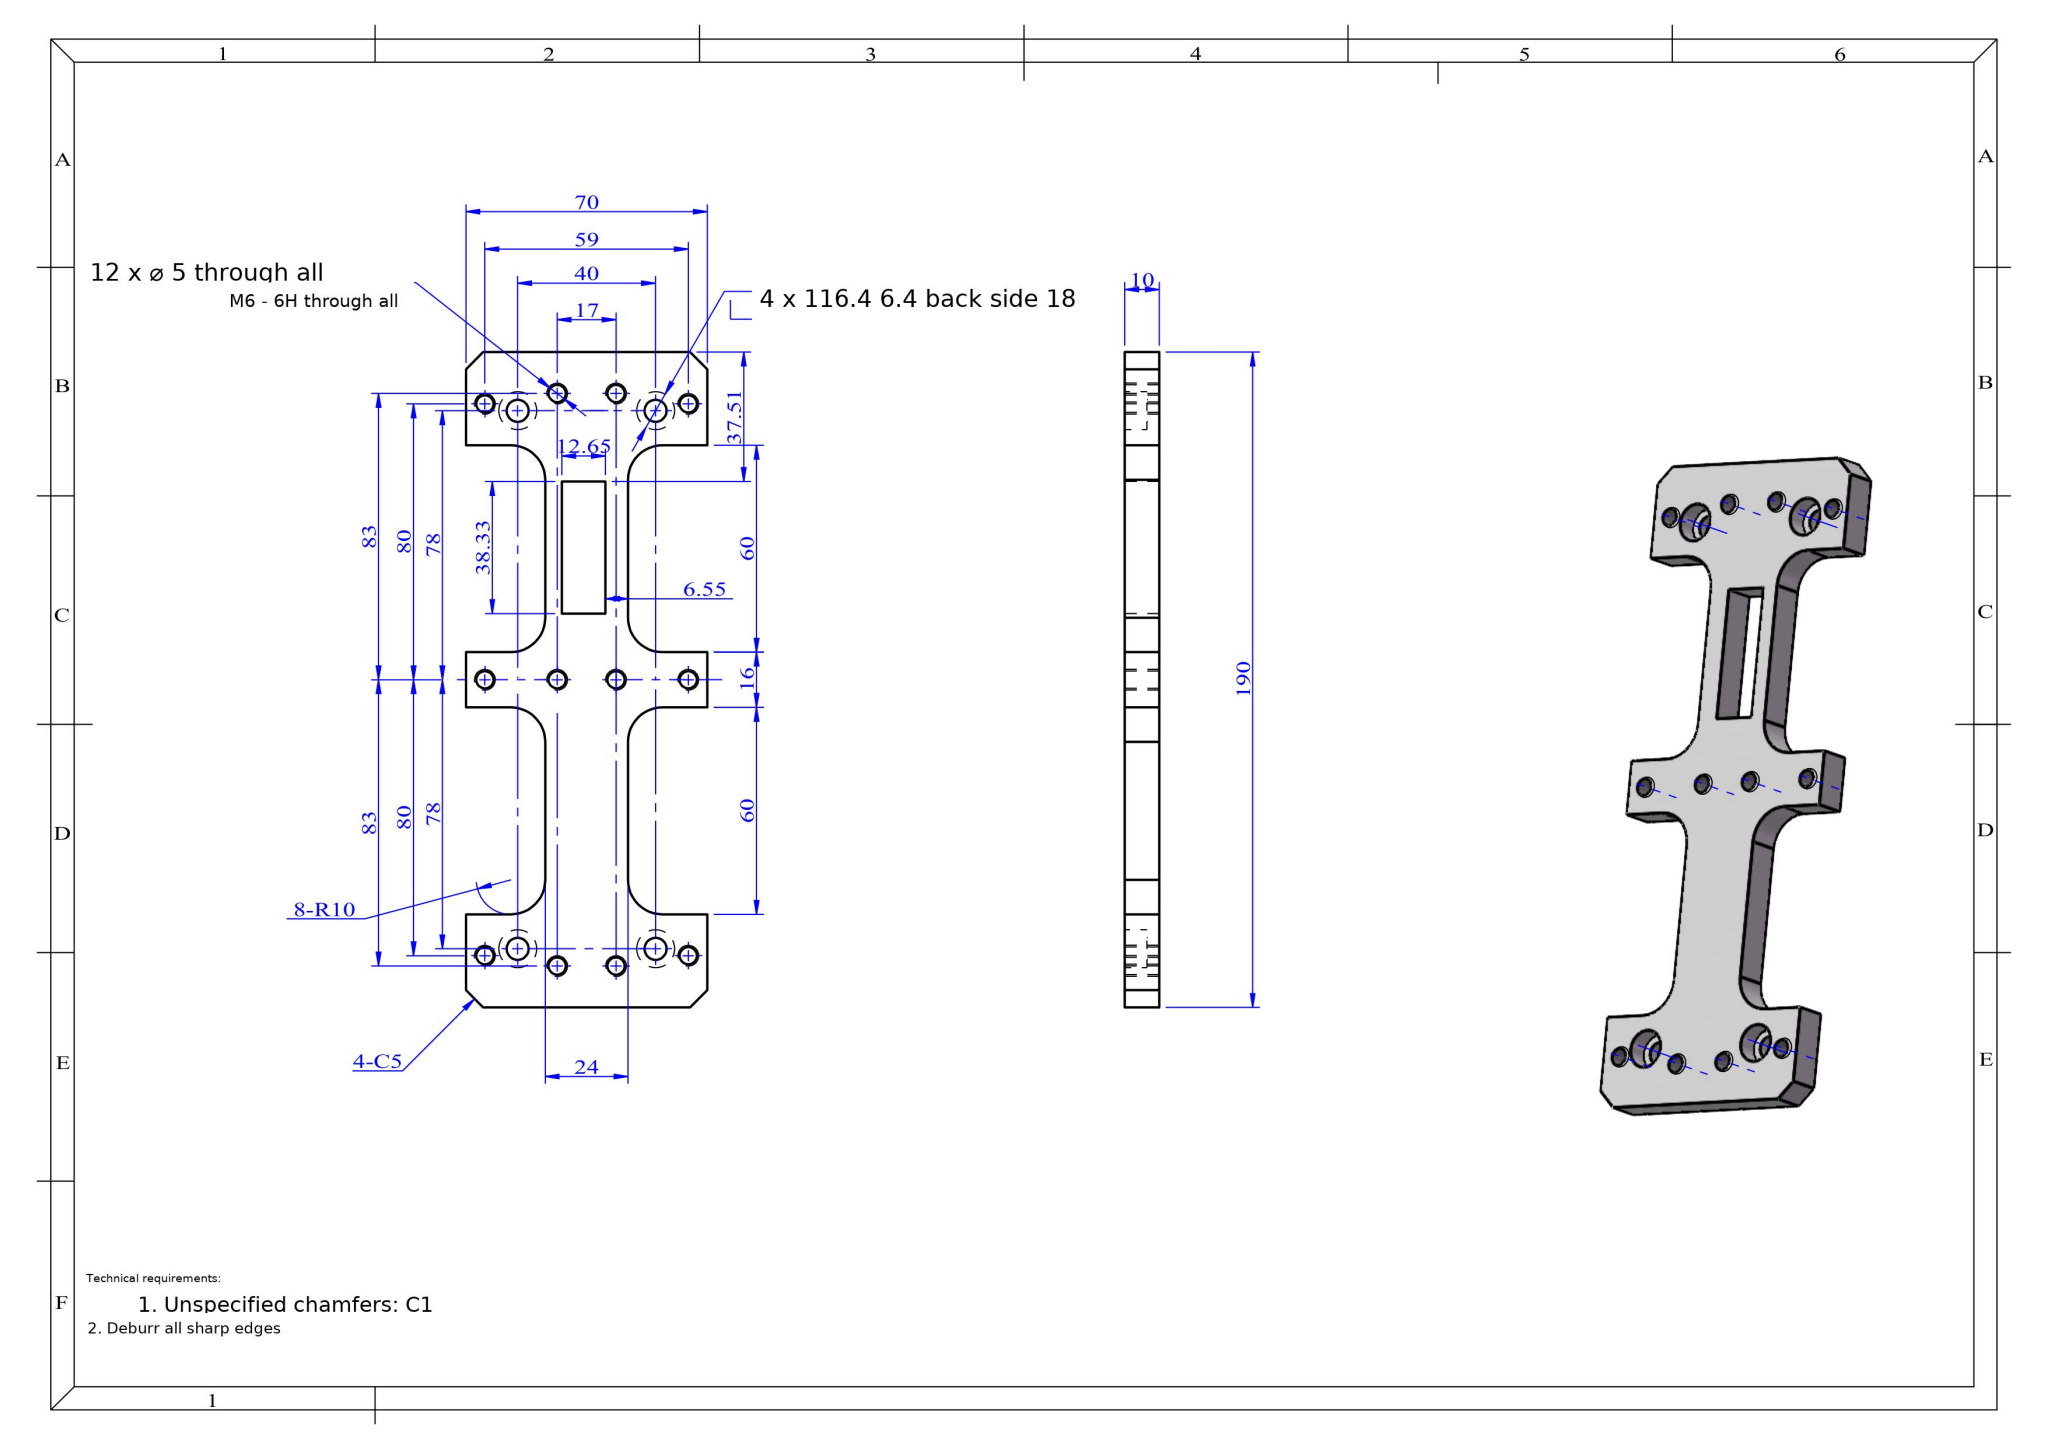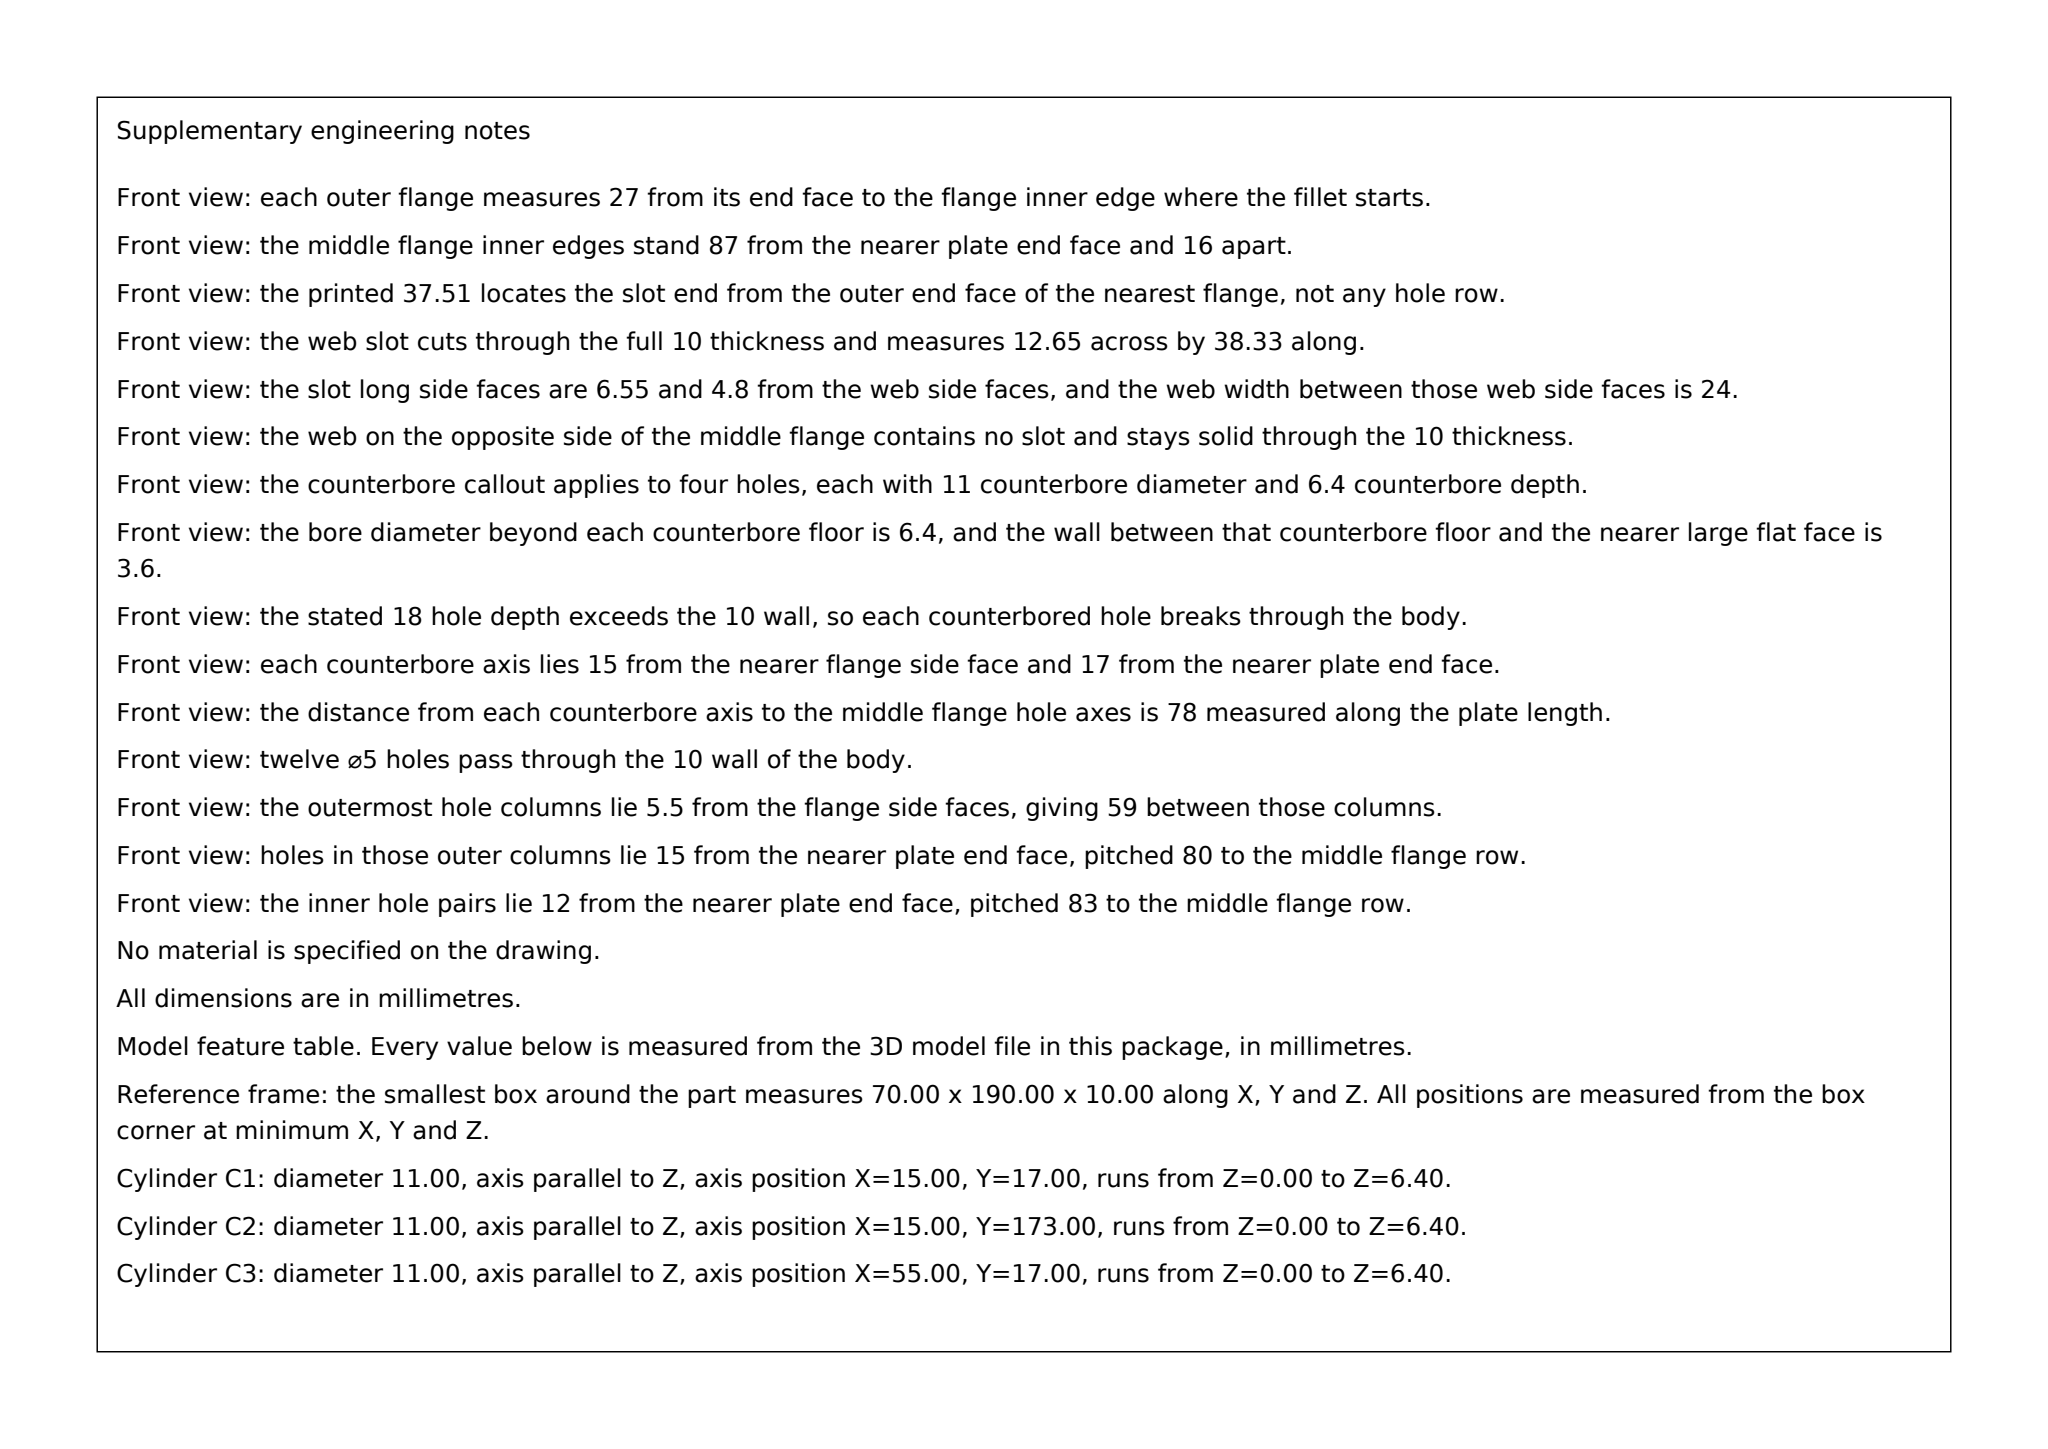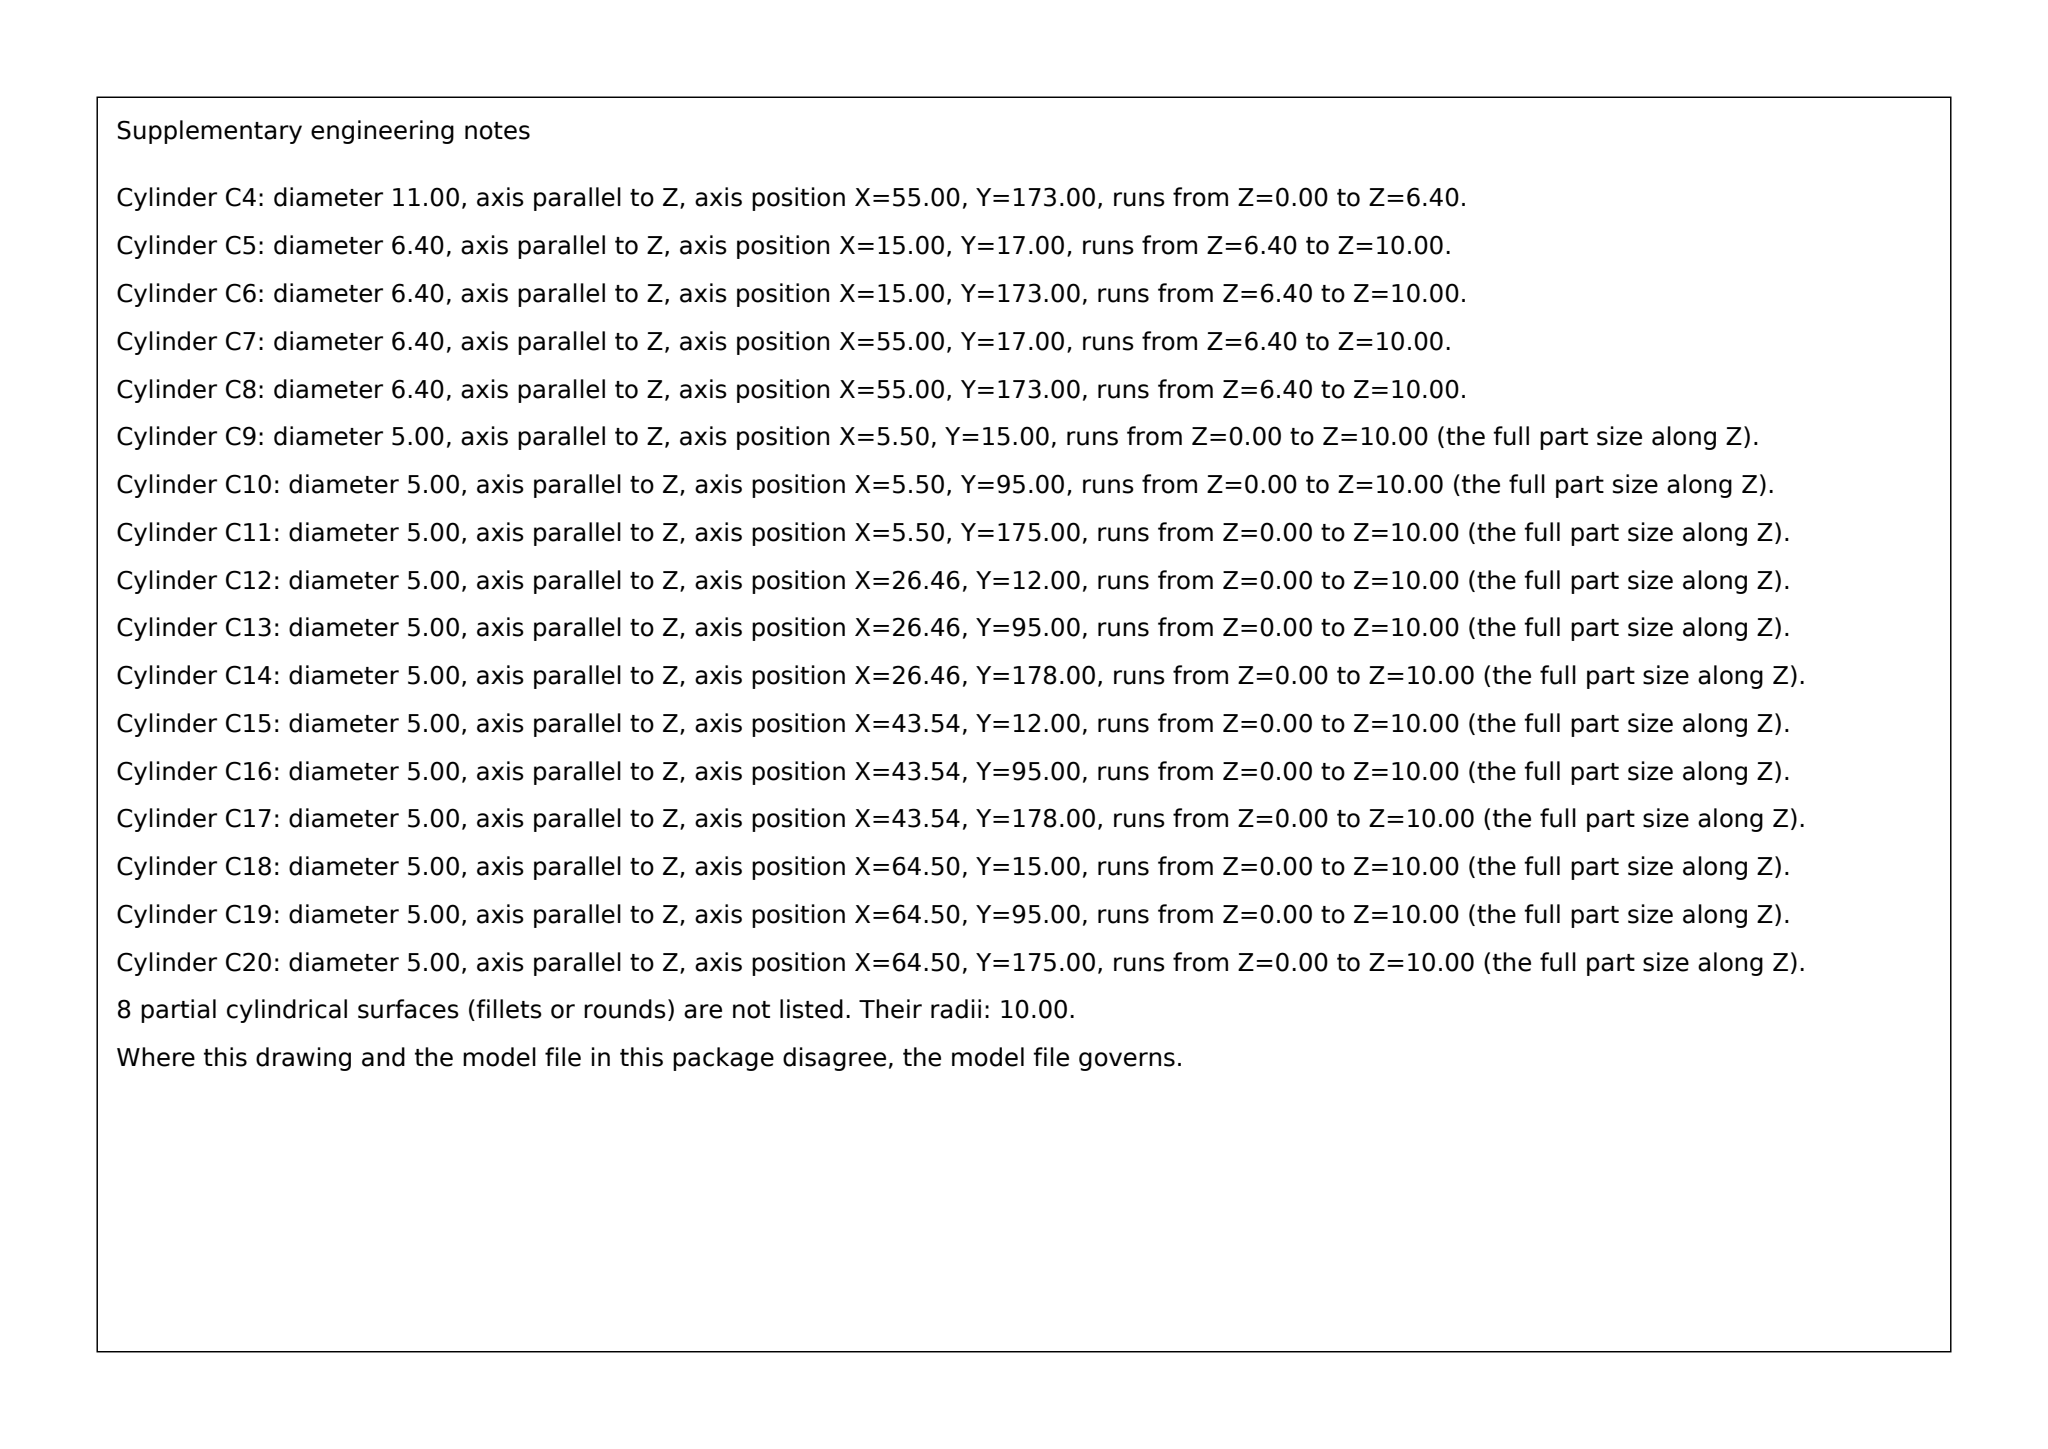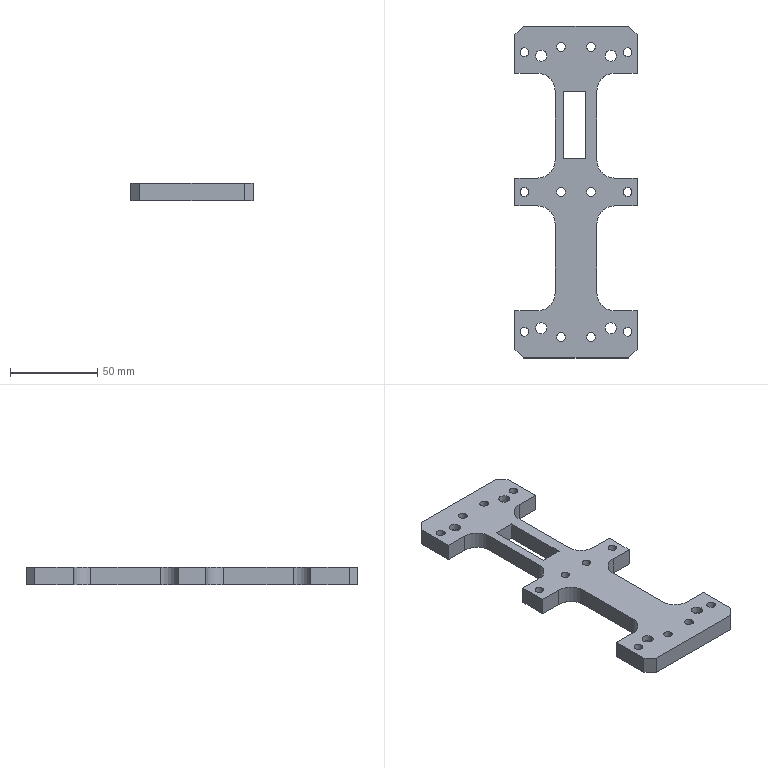Part | SolidWorks | mm | 1 solid | 82 faces | box 70 x 190 x 10 mm | volume 68917 mm3 | cylinder 48 | plane 34 | commonest cylinder face diameters 5 x24 11 x8 6.4 x8 20 x8
build123d program:
from build123d import *

# Parameters (mm, degrees)
SKETCH1_W                                       = 70
SKETCH1_H                                       = 190
BOSS_EXTRUDE1_DEPTH                             = 10
M6_HEX_SOCKET_HEAD_CAP_SCREW_CBORE1_D           = 6.4
M6_HEX_SOCKET_HEAD_CAP_SCREW_CBORE1_DEPTH       = 18
M6_HEX_SOCKET_HEAD_CAP_SCREW_CBORE1_CBORE_D     = 11
M6_HEX_SOCKET_HEAD_CAP_SCREW_CBORE1_CBORE_DEPTH = 6.4
M6_HEX_SOCKET_HEAD_CAP_SCREW_CBORE1_TIP         = 1.923
M6_TAPPED_HOLE1_D                               = 5
M6_TAPPED_HOLE2_D                               = 5
CHAMFER1_SIZE                                   = 5
SKETCH8_W                                       = 23
SKETCH8_H                                       = 60
CUT_EXTRUDE1_DEPTH                              = 203.731
FILLET1_R                                       = 10
SKETCH9_W                                       = 12.646
SKETCH9_H                                       = 38.328
CUT_EXTRUDE2_DEPTH                              = 44


with BuildPart() as part:
    # Sketch1 → Boss-Extrude1 (new body)
    with BuildSketch(Plane.XY):
        with Locations((35, 95)):
            Rectangle(SKETCH1_W, SKETCH1_H)
    extrude(amount=BOSS_EXTRUDE1_DEPTH)

    # M6 Hex Socket Head Cap Screw CBORE1
    with Locations(Plane(origin=(0, 0, 0), x_dir=(-1, 0, 0), z_dir=(0, 0, -1))):
        with Locations((-15, 173), (-55, 173), (-55, 17), (-15, 17)):
            CounterBoreHole(M6_HEX_SOCKET_HEAD_CAP_SCREW_CBORE1_D / 2, M6_HEX_SOCKET_HEAD_CAP_SCREW_CBORE1_CBORE_D / 2, M6_HEX_SOCKET_HEAD_CAP_SCREW_CBORE1_CBORE_DEPTH, depth=M6_HEX_SOCKET_HEAD_CAP_SCREW_CBORE1_DEPTH)
            with Locations((0, 0, -(M6_HEX_SOCKET_HEAD_CAP_SCREW_CBORE1_DEPTH + M6_HEX_SOCKET_HEAD_CAP_SCREW_CBORE1_TIP / 2))):  # 118° drill point
                Cone(0, M6_HEX_SOCKET_HEAD_CAP_SCREW_CBORE1_D / 2, M6_HEX_SOCKET_HEAD_CAP_SCREW_CBORE1_TIP, mode=Mode.SUBTRACT)

    # M6 Tapped Hole1 (through all)
    with Locations(Plane(origin=(0, 0, 0), x_dir=(-1, 0, 0), z_dir=(0, 0, -1))):
        with Locations((-43.536, 178), (-26.464, 178), (-43.536, 95), (-26.464, 95), (-43.536, 12), (-26.464, 12)):
            Hole(M6_TAPPED_HOLE1_D / 2)

    # M6 Tapped Hole2 (through all)
    with Locations(Plane(origin=(0, 0, 0), x_dir=(-1, 0, 0), z_dir=(0, 0, -1))):
        with Locations((-5.5, 175), (-5.5, 95), (-5.5, 15)):
            m6_tapped_hole2 = Hole(M6_TAPPED_HOLE2_D / 2)

    # Mirror1: M6 Tapped Hole2 across plane
    add(m6_tapped_hole2.mirror(Plane(origin=(35, 0, 0), x_dir=(0, 0, 1), z_dir=(1, 0, 0))), mode=Mode.SUBTRACT)

    # Chamfer1
    chamfer1_edges = [part.edges().sort_by_distance(p)[0] for p in [
        (0, 190, 5),
        (70, 190, 5),
        (70, 0, 5),
        (0, 0, 5),
    ]]
    chamfer(chamfer1_edges, length=CHAMFER1_SIZE)

    # Sketch8 → Cut-Extrude1 (cut, through all)
    with BuildSketch(Plane(origin=(0, 0, 0), x_dir=(-1, 0, 0), z_dir=(0, 0, -1))):
        with Locations((-11.5, 133)):
            Rectangle(SKETCH8_W, SKETCH8_H)
        with Locations((-58.5, 133)):
            Rectangle(SKETCH8_W, SKETCH8_H)
        with Locations((-58.5, 57)):
            Rectangle(SKETCH8_W, SKETCH8_H)
        with Locations((-11.5, 57)):
            Rectangle(SKETCH8_W, SKETCH8_H)
    extrude(amount=-CUT_EXTRUDE1_DEPTH, mode=Mode.SUBTRACT)

    # Fillet1
    fillet1_edges = [part.edges().sort_by_distance(p)[0] for p in [
        (23, 103, 5),
        (23, 163, 5),
        (47, 163, 5),
        (47, 103, 5),
        (47, 87, 5),
        (47, 27, 5),
        (23, 27, 5),
        (23, 87, 5),
    ]]
    fillet(fillet1_edges, radius=FILLET1_R)

    # Sketch9 → Cut-Extrude2 (cut)
    with BuildSketch(Plane(origin=(0, 0, 0), x_dir=(-1, 0, 0), z_dir=(0, 0, -1))):
        with Locations((-34.124, 133.328)):
            Rectangle(SKETCH9_W, SKETCH9_H)
    extrude(amount=-CUT_EXTRUDE2_DEPTH, mode=Mode.SUBTRACT)


solid = part.part